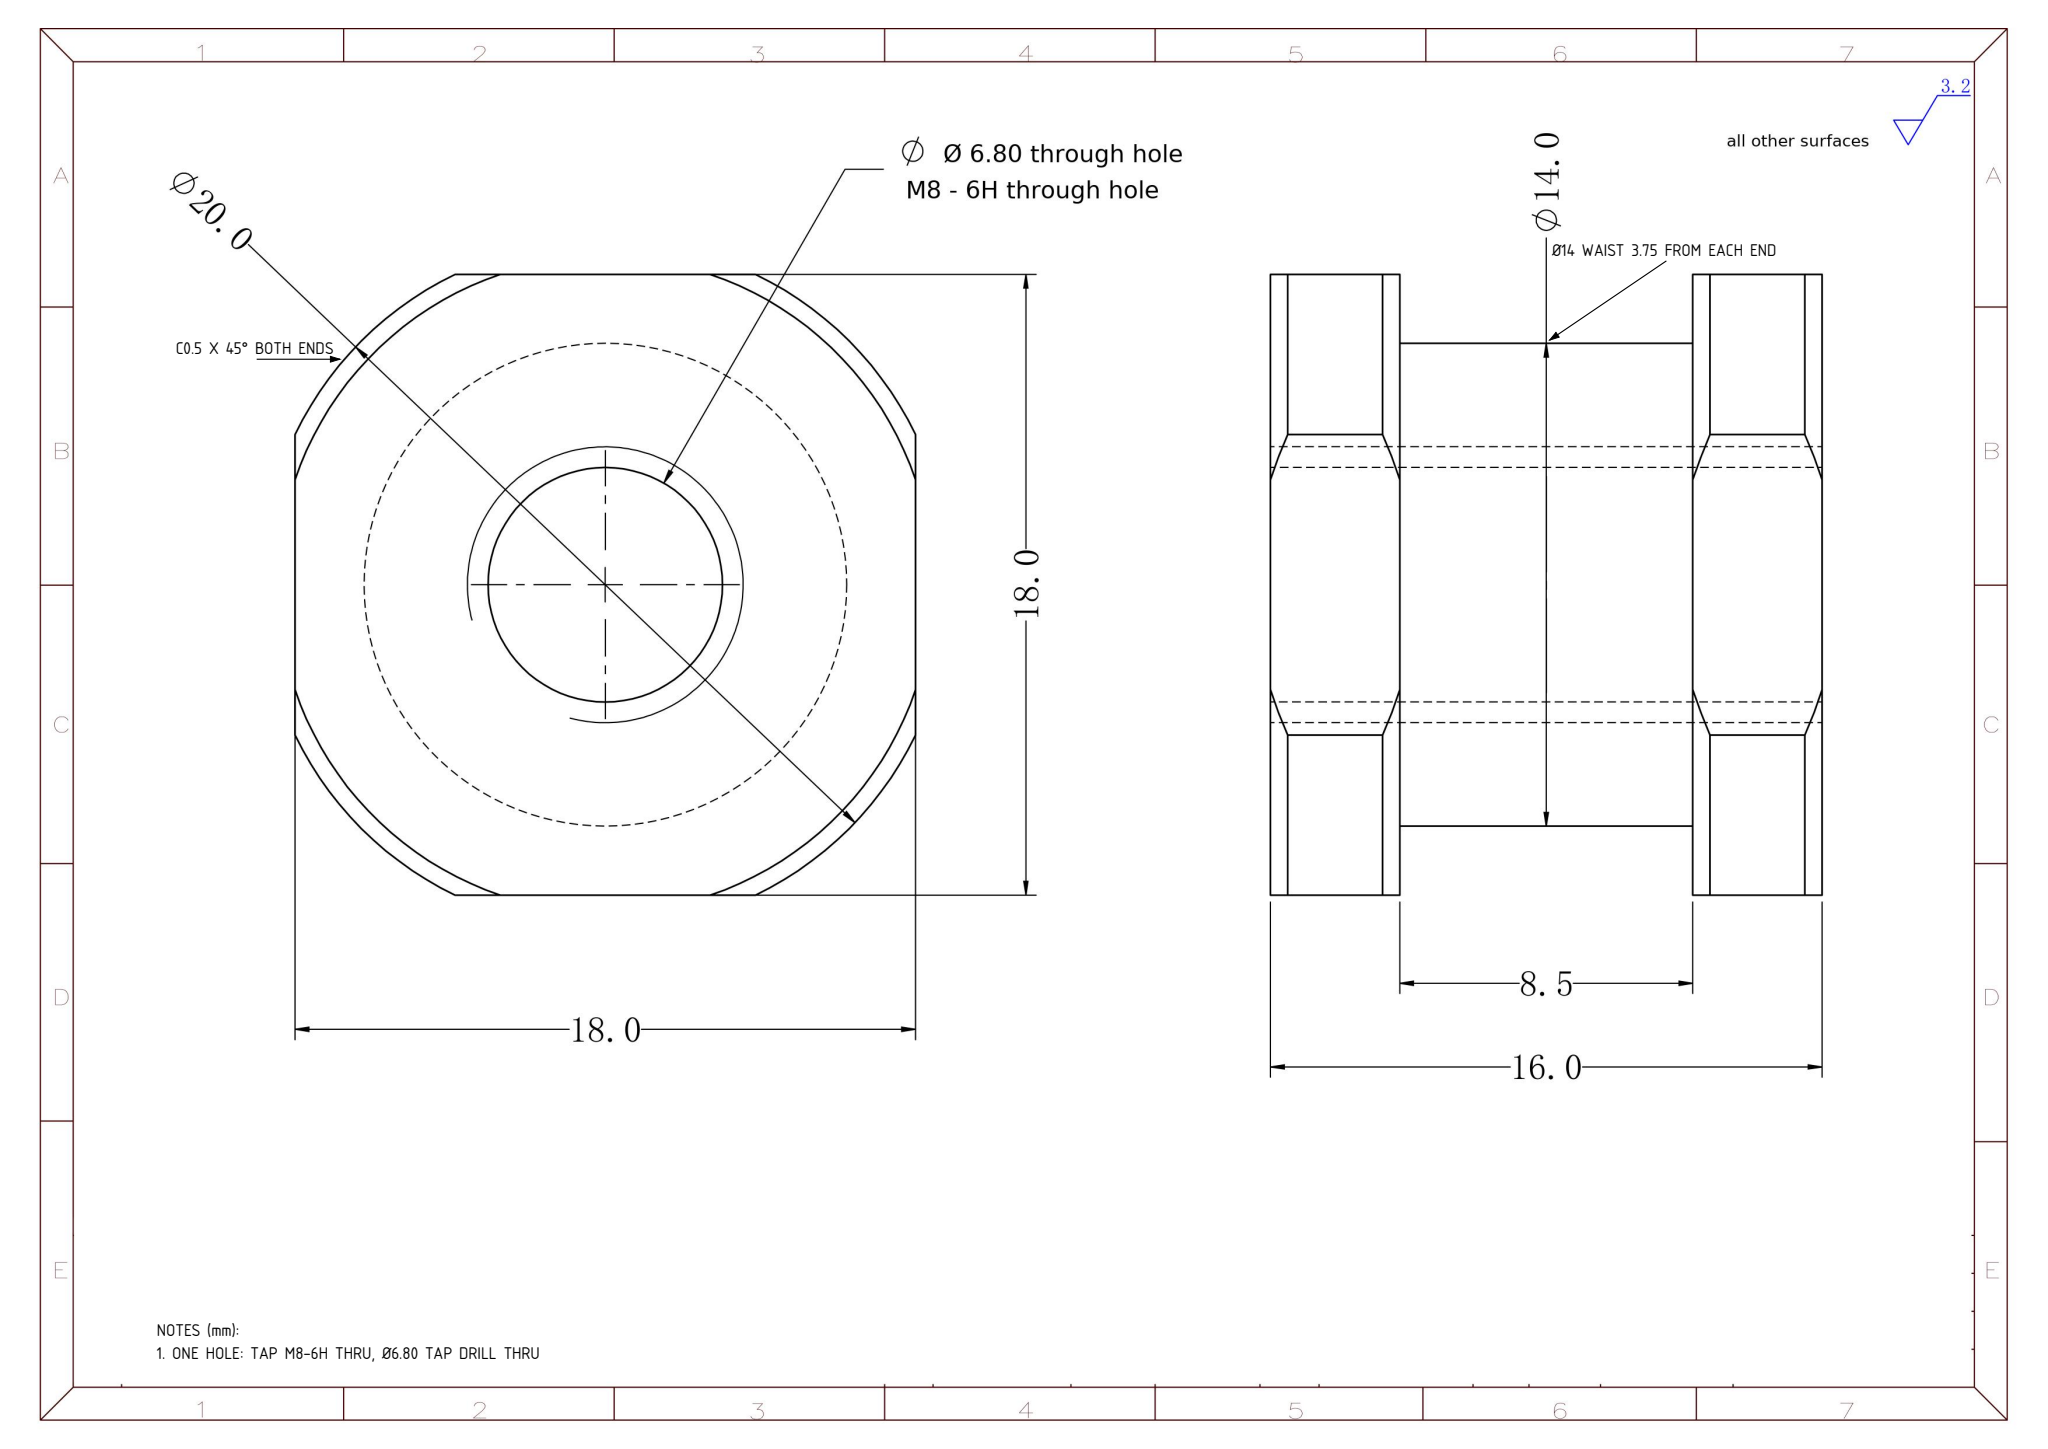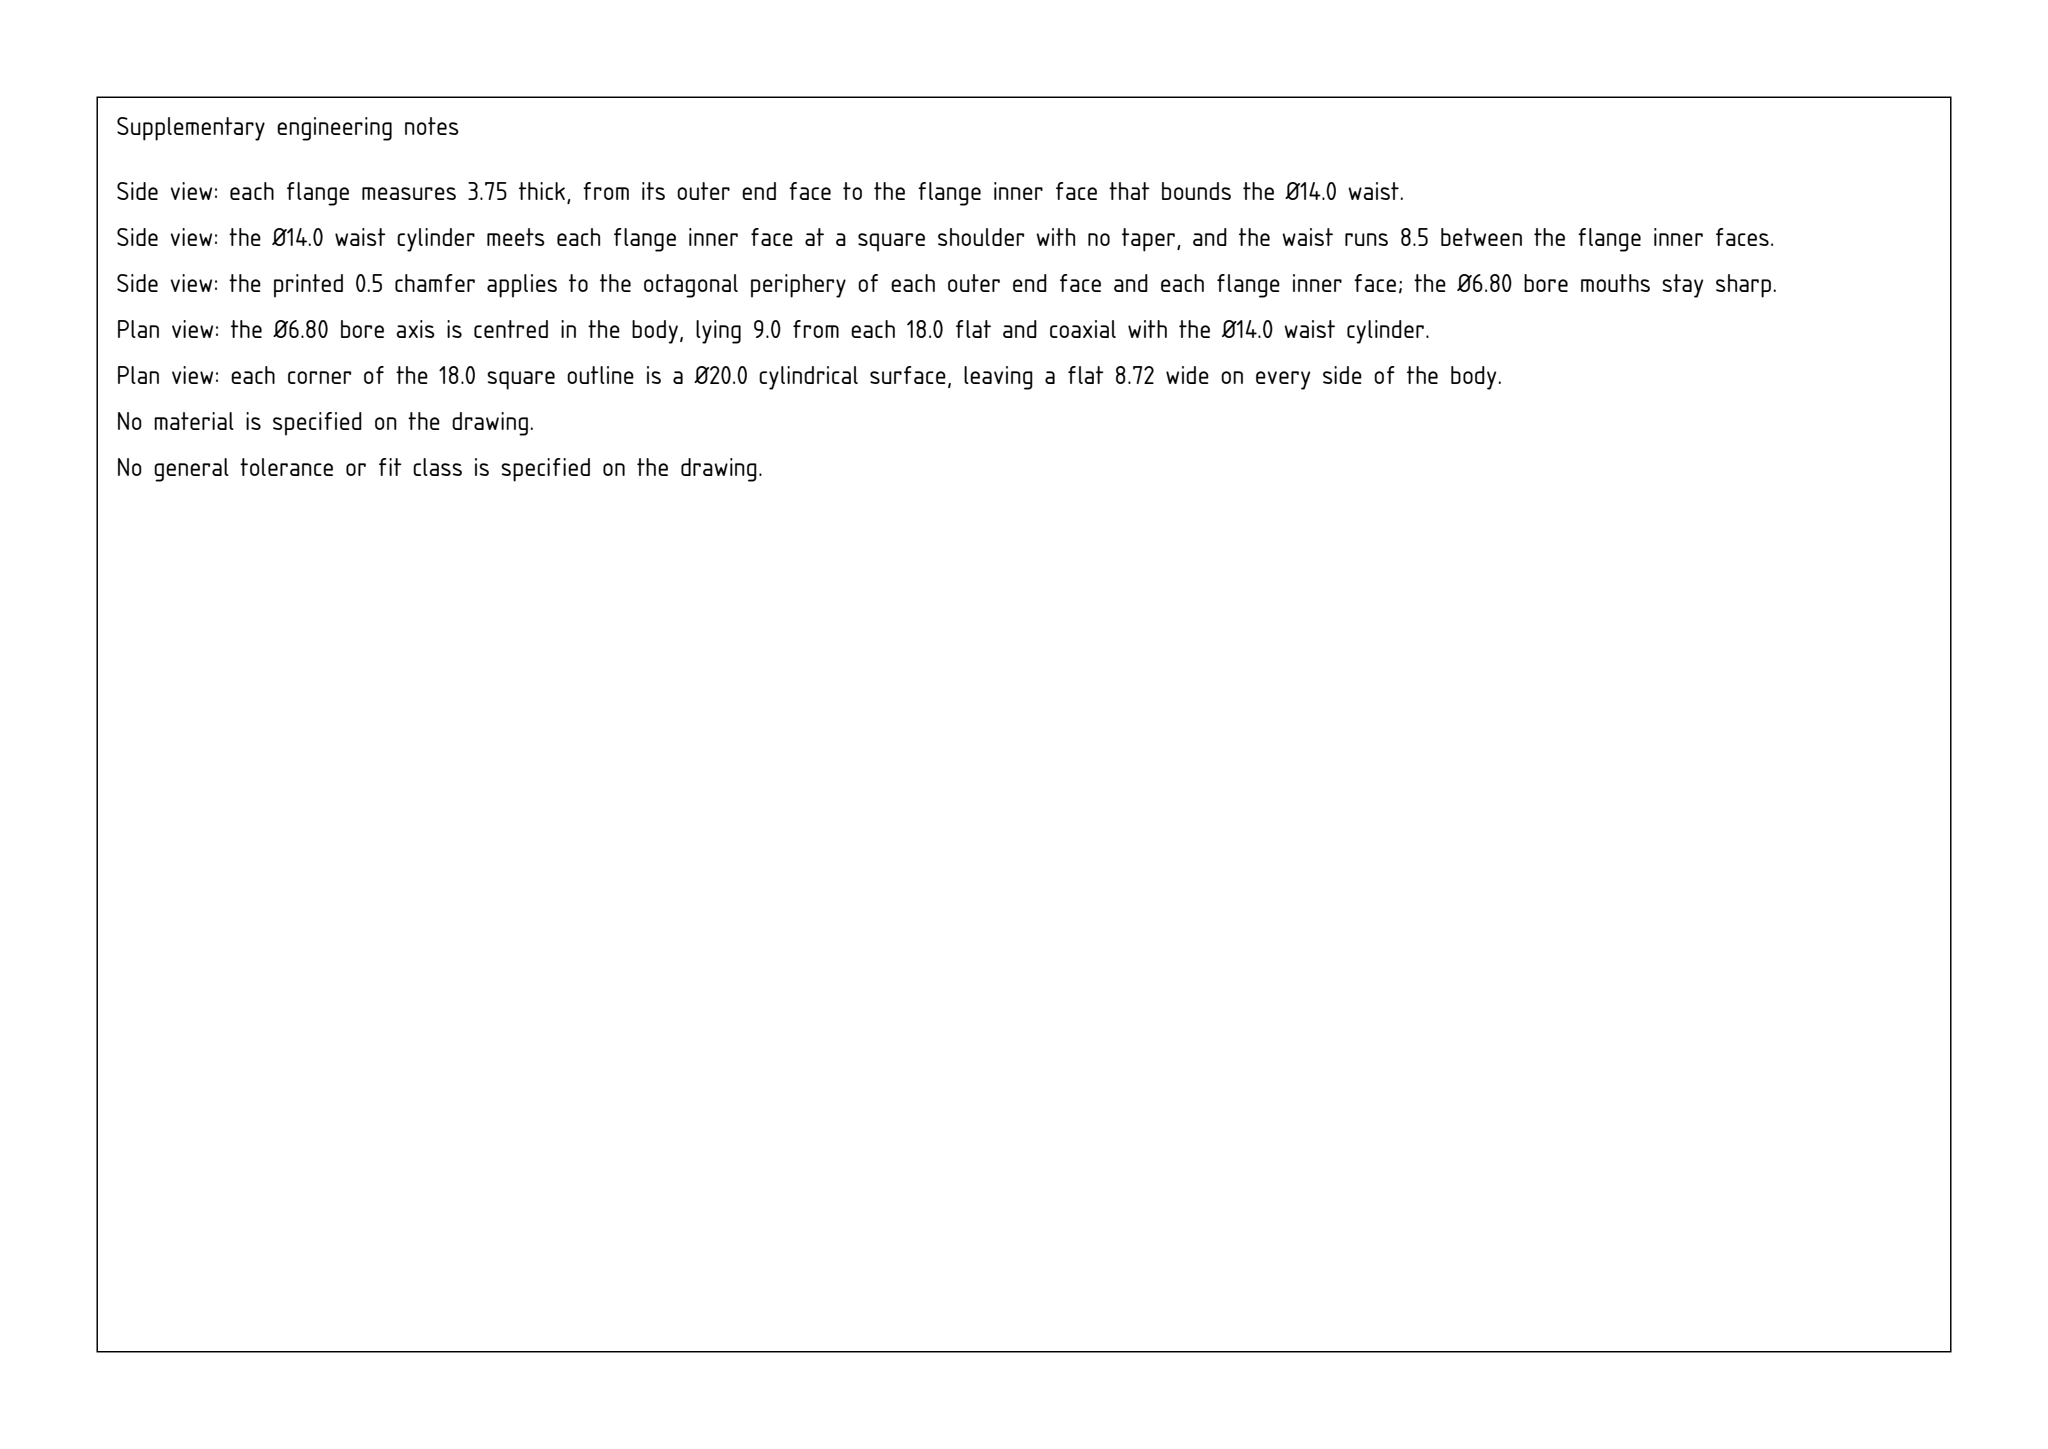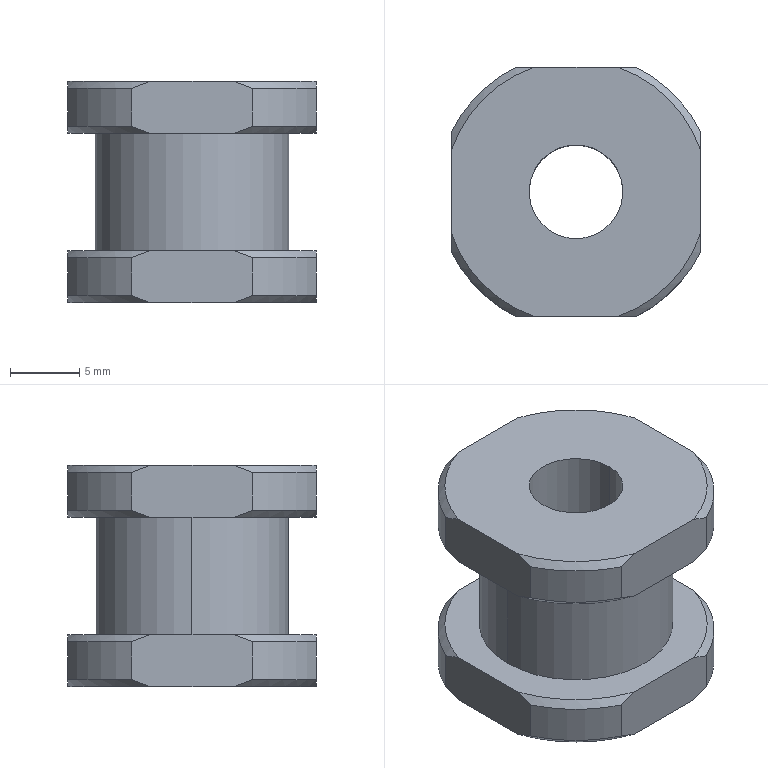Part | SolidWorks | mm | 1 solid | 40 faces | box 18 x 18 x 16 mm | volume 2893 mm3 | cone 16 | cylinder 12 | plane 12 | commonest cylinder face diameters 20 x8 6.8 x2 14 x2
Drawing notes:
CHAMFER 0.5 X 45° ON Ø20 CORNER ARCS, BOTH ENDS (Ø20 TO Ø19) | from the solid: cones included angle 90.0 between ref_dia 20.0 and 19.0, 8 each end; Ø20 cyl len 2.75 at z 0-2.75 and 13.25-16.0
Ø14.0 x 8.5 WAIST SYM ABOUT MID-LENGTH; 3.75 FROM EACH END | from the solid: Ø14 cyl z=3.75 to 12.25, len 8.5 in 16.0 overall; planes z=3.75,12.25
ONE HOLE: TAP M8-6H THRU, Ø6.80 TAP DRILL THRU | from the solid: single Ø6.80 z-axis cyl at (9.47,9.47), length 16.0 thru
build123d program:
from build123d import *

# Parameters (mm, degrees)
SKETCH1_R           = 10
BOSS_EXTRUDE1_DEPTH = 8
SKETCH2_R           = 10
SKETCH2_R_2         = 7
CUT_EXTRUDE1_DEPTH  = 4.25
M8_TAPPED_HOLE1_D   = 6.8
CHAMFER1_SIZE       = 0.5
SKETCH5_W           = 25
SKETCH5_H           = 25
SKETCH5_W_2         = 18
SKETCH5_H_2         = 18
CUT_EXTRUDE2_DEPTH  = 22.354


with BuildPart() as part:
    # Sketch1 → Boss-Extrude1 (new, symmetric)
    with BuildSketch(Plane.XY):
        Circle(SKETCH1_R)
    extrude(amount=BOSS_EXTRUDE1_DEPTH, both=True)

    # Sketch2 → Cut-Extrude1 (cut, symmetric)
    with BuildSketch(Plane.XY):
        Circle(SKETCH2_R)
        Circle(SKETCH2_R_2, mode=Mode.SUBTRACT)
    extrude(amount=CUT_EXTRUDE1_DEPTH, both=True, mode=Mode.SUBTRACT)

    # M8 Tapped Hole1 (through all)
    with Locations(Plane.XY.offset(8)):
        with Locations((0, 0)):
            Hole(M8_TAPPED_HOLE1_D / 2)

    # Chamfer1
    chamfer1_edges = [part.edges().sort_by_distance(p)[0] for p in [
        (-10, 0, -8),
        (-10, 0, 8),
        (-10, 0, -4.25),
        (-10, 0, 4.25),
    ]]
    chamfer(chamfer1_edges, length=CHAMFER1_SIZE)

    # Sketch5 → Cut-Extrude2 (cut, through all)
    with BuildSketch(Plane(origin=(0, 0, -8), x_dir=(-1, 0, 0), z_dir=(0, 0, -1))):
        Rectangle(SKETCH5_W, SKETCH5_H)
        Rectangle(SKETCH5_W_2, SKETCH5_H_2, mode=Mode.SUBTRACT)
    extrude(amount=-CUT_EXTRUDE2_DEPTH, mode=Mode.SUBTRACT)


solid = part.part